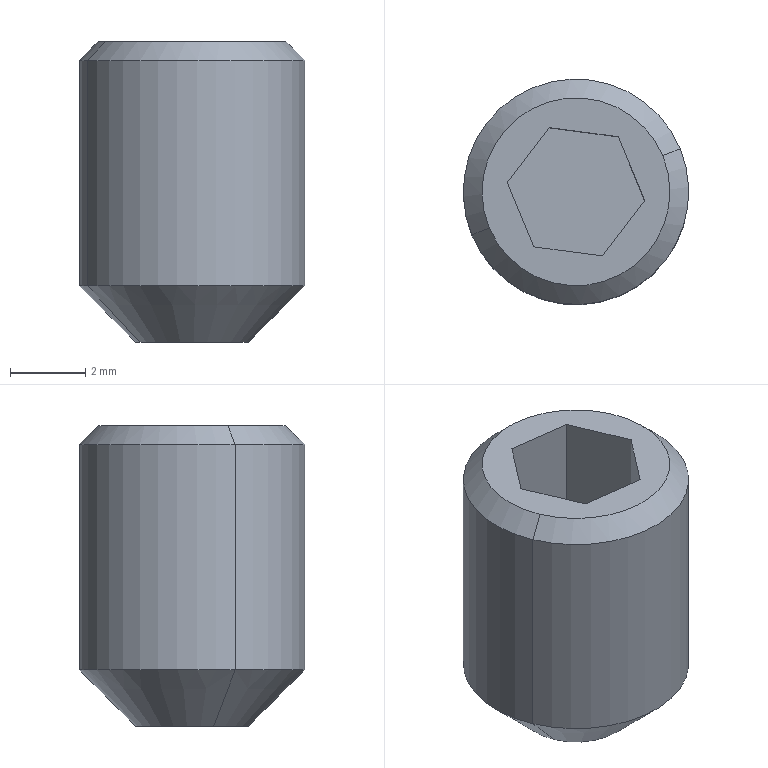Component | SolidWorks | M6x8GrubScrew-3 | 1 solid | 15 faces | box 6 x 6 x 8 mm | volume 171 mm3 | plane 9 | cone 4 | cylinder 2 | commonest cylinder face diameters 6 x2 | material #45
STEP:
#1=COLOUR_RGB('',0.7922,0.8196,0.9333);
#2=FILL_AREA_STYLE_COLOUR('',#1);
#3=FILL_AREA_STYLE('',(#2));
#4=SURFACE_STYLE_FILL_AREA(#3);
#5=SURFACE_SIDE_STYLE('',(#4));
#6=SURFACE_STYLE_USAGE(.BOTH.,#5);
#7=PRESENTATION_STYLE_ASSIGNMENT((#6));
#8=CARTESIAN_POINT('',(-3.53,0.5679,0.4724));
#9=VERTEX_POINT('',#8);
#10=CARTESIAN_POINT('',(-3.421,0.6132,0.4724));
#11=VERTEX_POINT('',#10);
#12=CARTESIAN_POINT('',(-3.476,0.5906,0.4724));
#13=DIRECTION('',(0.,-0.,-1.));
#14=DIRECTION('',(-0.9237,-0.383,0.));
#15=AXIS2_PLACEMENT_3D('',#12,#13,#14);
#16=CIRCLE('',#15,0.05906);
#17=EDGE_CURVE('',#9,#11,#16,.T.);
#18=ORIENTED_EDGE('',*,*,#17,.F.);
#19=CARTESIAN_POINT('',(-3.585,0.5453,0.5315));
#20=VERTEX_POINT('',#19);
#21=CARTESIAN_POINT('',(-3.585,0.5453,0.5315));
#22=DIRECTION('',(-0.6532,-0.2709,0.7071));
#23=VECTOR('',#22,39.37);
#24=LINE('',#21,#23);
#25=EDGE_CURVE('',#9,#20,#24,.T.);
#26=ORIENTED_EDGE('',*,*,#25,.T.);
#27=CARTESIAN_POINT('',(-3.367,0.6358,0.5315));
#28=VERTEX_POINT('',#27);
#29=CARTESIAN_POINT('',(-3.476,0.5906,0.5315));
#30=DIRECTION('',(0.,-0.,-1.));
#31=DIRECTION('',(-0.9237,-0.383,0.));
#32=AXIS2_PLACEMENT_3D('',#29,#30,#31);
#33=CIRCLE('',#32,0.1181);
#34=EDGE_CURVE('',#20,#28,#33,.T.);
#35=ORIENTED_EDGE('',*,*,#34,.T.);
#36=CARTESIAN_POINT('',(-3.367,0.6358,0.5315));
#37=DIRECTION('',(0.6532,0.2709,0.7071));
#38=VECTOR('',#37,39.37);
#39=LINE('',#36,#38);
#40=EDGE_CURVE('',#11,#28,#39,.T.);
#41=ORIENTED_EDGE('',*,*,#40,.F.);
#42=EDGE_LOOP('',(#18,#26,#35,#41));
#43=FACE_OUTER_BOUND('',#42,.T.);
#44=CARTESIAN_POINT('',(-3.476,0.5906,0.5315));
#45=DIRECTION('',(-0.,0.,1.));
#46=DIRECTION('',(0.9237,0.383,0.));
#47=AXIS2_PLACEMENT_3D('',#44,#45,#46);
#48=CONICAL_SURFACE('',#47,0.1181,0.7854);
#49=ADVANCED_FACE('',(#43),#48,.T.);
#50=CARTESIAN_POINT('',(-3.585,0.5453,0.7677));
#51=VERTEX_POINT('',#50);
#52=CARTESIAN_POINT('',(-3.367,0.6358,0.7677));
#53=VERTEX_POINT('',#52);
#54=CARTESIAN_POINT('',(-3.476,0.5906,0.7677));
#55=DIRECTION('',(0.,-0.,-1.));
#56=DIRECTION('',(-0.9237,-0.383,0.));
#57=AXIS2_PLACEMENT_3D('',#54,#55,#56);
#58=CIRCLE('',#57,0.1181);
#59=EDGE_CURVE('',#51,#53,#58,.T.);
#60=ORIENTED_EDGE('',*,*,#59,.T.);
#61=CARTESIAN_POINT('',(-3.367,0.6358,0.4724));
#62=DIRECTION('',(0.,-0.,-1.));
#63=VECTOR('',#62,39.37);
#64=LINE('',#61,#63);
#65=EDGE_CURVE('',#53,#28,#64,.T.);
#66=ORIENTED_EDGE('',*,*,#65,.T.);
#67=ORIENTED_EDGE('',*,*,#34,.F.);
#68=CARTESIAN_POINT('',(-3.585,0.5453,0.4724));
#69=DIRECTION('',(0.,-0.,-1.));
#70=VECTOR('',#69,39.37);
#71=LINE('',#68,#70);
#72=EDGE_CURVE('',#51,#20,#71,.T.);
#73=ORIENTED_EDGE('',*,*,#72,.F.);
#74=EDGE_LOOP('',(#60,#66,#67,#73));
#75=FACE_OUTER_BOUND('',#74,.T.);
#76=CARTESIAN_POINT('',(-3.476,0.5906,0.4724));
#77=DIRECTION('',(0.,-0.,-1.));
#78=DIRECTION('',(-0.9237,-0.383,0.));
#79=AXIS2_PLACEMENT_3D('',#76,#77,#78);
#80=CYLINDRICAL_SURFACE('',#79,0.1181);
#81=ADVANCED_FACE('',(#75),#80,.T.);
#82=CARTESIAN_POINT('',(-3.567,0.5528,0.7874));
#83=VERTEX_POINT('',#82);
#84=CARTESIAN_POINT('',(-3.385,0.6283,0.7874));
#85=VERTEX_POINT('',#84);
#86=CARTESIAN_POINT('',(-3.476,0.5906,0.7874));
#87=DIRECTION('',(0.,-0.,-1.));
#88=DIRECTION('',(-0.9237,-0.383,0.));
#89=AXIS2_PLACEMENT_3D('',#86,#87,#88);
#90=CIRCLE('',#89,0.09843);
#91=EDGE_CURVE('',#83,#85,#90,.T.);
#92=ORIENTED_EDGE('',*,*,#91,.T.);
#93=CARTESIAN_POINT('',(-3.385,0.6283,0.7874));
#94=DIRECTION('',(0.6532,0.2709,-0.7071));
#95=VECTOR('',#94,39.37);
#96=LINE('',#93,#95);
#97=EDGE_CURVE('',#85,#53,#96,.T.);
#98=ORIENTED_EDGE('',*,*,#97,.T.);
#99=ORIENTED_EDGE('',*,*,#59,.F.);
#100=CARTESIAN_POINT('',(-3.567,0.5528,0.7874));
#101=DIRECTION('',(-0.6532,-0.2709,-0.7071));
#102=VECTOR('',#101,39.37);
#103=LINE('',#100,#102);
#104=EDGE_CURVE('',#83,#51,#103,.T.);
#105=ORIENTED_EDGE('',*,*,#104,.F.);
#106=EDGE_LOOP('',(#92,#98,#99,#105));
#107=FACE_OUTER_BOUND('',#106,.T.);
#108=CARTESIAN_POINT('',(-3.476,0.5906,0.7874));
#109=DIRECTION('',(0.,-0.,-1.));
#110=DIRECTION('',(-0.9237,-0.383,0.));
#111=AXIS2_PLACEMENT_3D('',#108,#109,#110);
#112=CONICAL_SURFACE('',#111,0.09843,0.7854);
#113=ADVANCED_FACE('',(#107),#112,.T.);
#114=CARTESIAN_POINT('',(-3.504,0.6577,0.7874));
#115=VERTEX_POINT('',#114);
#116=CARTESIAN_POINT('',(-3.548,0.6,0.7874));
#117=VERTEX_POINT('',#116);
#118=CARTESIAN_POINT('',(-3.504,0.6577,0.7874));
#119=DIRECTION('',(-0.6084,-0.7936,-0.));
#120=VECTOR('',#119,39.37);
#121=LINE('',#118,#120);
#122=EDGE_CURVE('',#115,#117,#121,.T.);
#123=ORIENTED_EDGE('',*,*,#122,.F.);
#124=CARTESIAN_POINT('',(-3.432,0.6483,0.7874));
#125=VERTEX_POINT('',#124);
#126=CARTESIAN_POINT('',(-3.432,0.6483,0.7874));
#127=DIRECTION('',(-0.9915,0.1301,-0.));
#128=VECTOR('',#127,39.37);
#129=LINE('',#126,#128);
#130=EDGE_CURVE('',#125,#115,#129,.T.);
#131=ORIENTED_EDGE('',*,*,#130,.F.);
#132=CARTESIAN_POINT('',(-3.404,0.5811,0.7874));
#133=VERTEX_POINT('',#132);
#134=CARTESIAN_POINT('',(-3.404,0.5811,0.7874));
#135=DIRECTION('',(-0.383,0.9237,-0.));
#136=VECTOR('',#135,39.37);
#137=LINE('',#134,#136);
#138=EDGE_CURVE('',#133,#125,#137,.T.);
#139=ORIENTED_EDGE('',*,*,#138,.F.);
#140=CARTESIAN_POINT('',(-3.448,0.5234,0.7874));
#141=VERTEX_POINT('',#140);
#142=CARTESIAN_POINT('',(-3.448,0.5234,0.7874));
#143=DIRECTION('',(0.6084,0.7936,0.));
#144=VECTOR('',#143,39.37);
#145=LINE('',#142,#144);
#146=EDGE_CURVE('',#141,#133,#145,.T.);
#147=ORIENTED_EDGE('',*,*,#146,.F.);
#148=CARTESIAN_POINT('',(-3.52,0.5328,0.7874));
#149=VERTEX_POINT('',#148);
#150=CARTESIAN_POINT('',(-3.52,0.5328,0.7874));
#151=DIRECTION('',(0.9915,-0.1301,0.));
#152=VECTOR('',#151,39.37);
#153=LINE('',#150,#152);
#154=EDGE_CURVE('',#149,#141,#153,.T.);
#155=ORIENTED_EDGE('',*,*,#154,.F.);
#156=CARTESIAN_POINT('',(-3.548,0.6,0.7874));
#157=DIRECTION('',(0.383,-0.9237,0.));
#158=VECTOR('',#157,39.37);
#159=LINE('',#156,#158);
#160=EDGE_CURVE('',#117,#149,#159,.T.);
#161=ORIENTED_EDGE('',*,*,#160,.F.);
#162=EDGE_LOOP('',(#123,#131,#139,#147,#155,#161));
#163=FACE_BOUND('',#162,.T.);
#164=ORIENTED_EDGE('',*,*,#91,.F.);
#165=CARTESIAN_POINT('',(-3.476,0.5906,0.7874));
#166=DIRECTION('',(0.,-0.,-1.));
#167=DIRECTION('',(-0.9237,-0.383,0.));
#168=AXIS2_PLACEMENT_3D('',#165,#166,#167);
#169=CIRCLE('',#168,0.09843);
#170=EDGE_CURVE('',#85,#83,#169,.T.);
#171=ORIENTED_EDGE('',*,*,#170,.F.);
#172=EDGE_LOOP('',(#164,#171));
#173=FACE_OUTER_BOUND('',#172,.T.);
#174=CARTESIAN_POINT('',(-3.476,0.5906,0.7874));
#175=DIRECTION('',(0.,-0.,-1.));
#176=DIRECTION('',(-0.9237,-0.383,-0.));
#177=AXIS2_PLACEMENT_3D('',#174,#175,#176);
#178=PLANE('',#177);
#179=ADVANCED_FACE('',(#163,#173),#178,.F.);
#180=ORIENTED_EDGE('',*,*,#97,.F.);
#181=ORIENTED_EDGE('',*,*,#170,.T.);
#182=ORIENTED_EDGE('',*,*,#104,.T.);
#183=CARTESIAN_POINT('',(-3.476,0.5906,0.7677));
#184=DIRECTION('',(0.,-0.,-1.));
#185=DIRECTION('',(-0.9237,-0.383,0.));
#186=AXIS2_PLACEMENT_3D('',#183,#184,#185);
#187=CIRCLE('',#186,0.1181);
#188=EDGE_CURVE('',#53,#51,#187,.T.);
#189=ORIENTED_EDGE('',*,*,#188,.F.);
#190=EDGE_LOOP('',(#180,#181,#182,#189));
#191=FACE_OUTER_BOUND('',#190,.T.);
#192=CARTESIAN_POINT('',(-3.476,0.5906,0.7874));
#193=DIRECTION('',(0.,-0.,-1.));
#194=DIRECTION('',(-0.9237,-0.383,0.));
#195=AXIS2_PLACEMENT_3D('',#192,#193,#194);
#196=CONICAL_SURFACE('',#195,0.09843,0.7854);
#197=ADVANCED_FACE('',(#191),#196,.T.);
#198=ORIENTED_EDGE('',*,*,#65,.F.);
#199=ORIENTED_EDGE('',*,*,#188,.T.);
#200=ORIENTED_EDGE('',*,*,#72,.T.);
#201=CARTESIAN_POINT('',(-3.476,0.5906,0.5315));
#202=DIRECTION('',(0.,-0.,-1.));
#203=DIRECTION('',(-0.9237,-0.383,0.));
#204=AXIS2_PLACEMENT_3D('',#201,#202,#203);
#205=CIRCLE('',#204,0.1181);
#206=EDGE_CURVE('',#28,#20,#205,.T.);
#207=ORIENTED_EDGE('',*,*,#206,.F.);
#208=EDGE_LOOP('',(#198,#199,#200,#207));
#209=FACE_OUTER_BOUND('',#208,.T.);
#210=CARTESIAN_POINT('',(-3.476,0.5906,0.4724));
#211=DIRECTION('',(0.,-0.,-1.));
#212=DIRECTION('',(-0.9237,-0.383,0.));
#213=AXIS2_PLACEMENT_3D('',#210,#211,#212);
#214=CYLINDRICAL_SURFACE('',#213,0.1181);
#215=ADVANCED_FACE('',(#209),#214,.T.);
#216=ORIENTED_EDGE('',*,*,#25,.F.);
#217=CARTESIAN_POINT('',(-3.476,0.5906,0.4724));
#218=DIRECTION('',(0.,-0.,-1.));
#219=DIRECTION('',(-0.9237,-0.383,0.));
#220=AXIS2_PLACEMENT_3D('',#217,#218,#219);
#221=CIRCLE('',#220,0.05906);
#222=EDGE_CURVE('',#11,#9,#221,.T.);
#223=ORIENTED_EDGE('',*,*,#222,.F.);
#224=ORIENTED_EDGE('',*,*,#40,.T.);
#225=ORIENTED_EDGE('',*,*,#206,.T.);
#226=EDGE_LOOP('',(#216,#223,#224,#225));
#227=FACE_OUTER_BOUND('',#226,.T.);
#228=CARTESIAN_POINT('',(-3.476,0.5906,0.5315));
#229=DIRECTION('',(-0.,0.,1.));
#230=DIRECTION('',(0.9237,0.383,0.));
#231=AXIS2_PLACEMENT_3D('',#228,#229,#230);
#232=CONICAL_SURFACE('',#231,0.1181,0.7854);
#233=ADVANCED_FACE('',(#227),#232,.T.);
#234=ORIENTED_EDGE('',*,*,#222,.T.);
#235=ORIENTED_EDGE('',*,*,#17,.T.);
#236=EDGE_LOOP('',(#234,#235));
#237=FACE_OUTER_BOUND('',#236,.T.);
#238=CARTESIAN_POINT('',(-3.421,0.6132,0.4724));
#239=DIRECTION('',(-0.,0.,1.));
#240=DIRECTION('',(0.9237,0.383,0.));
#241=AXIS2_PLACEMENT_3D('',#238,#239,#240);
#242=PLANE('',#241);
#243=ADVANCED_FACE('',(#237),#242,.F.);
#244=ORIENTED_EDGE('',*,*,#130,.T.);
#245=CARTESIAN_POINT('',(-3.504,0.6577,0.6299));
#246=VERTEX_POINT('',#245);
#247=CARTESIAN_POINT('',(-3.504,0.6577,0.6299));
#248=DIRECTION('',(-0.,0.,1.));
#249=VECTOR('',#248,39.37);
#250=LINE('',#247,#249);
#251=EDGE_CURVE('',#246,#115,#250,.T.);
#252=ORIENTED_EDGE('',*,*,#251,.F.);
#253=CARTESIAN_POINT('',(-3.432,0.6483,0.6299));
#254=VERTEX_POINT('',#253);
#255=CARTESIAN_POINT('',(-3.432,0.6483,0.6299));
#256=DIRECTION('',(-0.9915,0.1301,-0.));
#257=VECTOR('',#256,39.37);
#258=LINE('',#255,#257);
#259=EDGE_CURVE('',#254,#246,#258,.T.);
#260=ORIENTED_EDGE('',*,*,#259,.F.);
#261=CARTESIAN_POINT('',(-3.432,0.6483,0.6299));
#262=DIRECTION('',(-0.,0.,1.));
#263=VECTOR('',#262,39.37);
#264=LINE('',#261,#263);
#265=EDGE_CURVE('',#254,#125,#264,.T.);
#266=ORIENTED_EDGE('',*,*,#265,.T.);
#267=EDGE_LOOP('',(#244,#252,#260,#266));
#268=FACE_OUTER_BOUND('',#267,.T.);
#269=CARTESIAN_POINT('',(-3.432,0.6483,0.6299));
#270=DIRECTION('',(0.1301,0.9915,-0.));
#271=DIRECTION('',(0.9915,-0.1301,0.));
#272=AXIS2_PLACEMENT_3D('',#269,#270,#271);
#273=PLANE('',#272);
#274=ADVANCED_FACE('',(#268),#273,.F.);
#275=ORIENTED_EDGE('',*,*,#138,.T.);
#276=ORIENTED_EDGE('',*,*,#265,.F.);
#277=CARTESIAN_POINT('',(-3.404,0.5811,0.6299));
#278=VERTEX_POINT('',#277);
#279=CARTESIAN_POINT('',(-3.404,0.5811,0.6299));
#280=DIRECTION('',(-0.383,0.9237,-0.));
#281=VECTOR('',#280,39.37);
#282=LINE('',#279,#281);
#283=EDGE_CURVE('',#278,#254,#282,.T.);
#284=ORIENTED_EDGE('',*,*,#283,.F.);
#285=CARTESIAN_POINT('',(-3.404,0.5811,0.6299));
#286=DIRECTION('',(-0.,0.,1.));
#287=VECTOR('',#286,39.37);
#288=LINE('',#285,#287);
#289=EDGE_CURVE('',#278,#133,#288,.T.);
#290=ORIENTED_EDGE('',*,*,#289,.T.);
#291=EDGE_LOOP('',(#275,#276,#284,#290));
#292=FACE_OUTER_BOUND('',#291,.T.);
#293=CARTESIAN_POINT('',(-3.404,0.5811,0.6299));
#294=DIRECTION('',(0.9237,0.383,0.));
#295=DIRECTION('',(0.383,-0.9237,0.));
#296=AXIS2_PLACEMENT_3D('',#293,#294,#295);
#297=PLANE('',#296);
#298=ADVANCED_FACE('',(#292),#297,.F.);
#299=ORIENTED_EDGE('',*,*,#146,.T.);
#300=ORIENTED_EDGE('',*,*,#289,.F.);
#301=CARTESIAN_POINT('',(-3.448,0.5234,0.6299));
#302=VERTEX_POINT('',#301);
#303=CARTESIAN_POINT('',(-3.448,0.5234,0.6299));
#304=DIRECTION('',(0.6084,0.7936,0.));
#305=VECTOR('',#304,39.37);
#306=LINE('',#303,#305);
#307=EDGE_CURVE('',#302,#278,#306,.T.);
#308=ORIENTED_EDGE('',*,*,#307,.F.);
#309=CARTESIAN_POINT('',(-3.448,0.5234,0.6299));
#310=DIRECTION('',(-0.,0.,1.));
#311=VECTOR('',#310,39.37);
#312=LINE('',#309,#311);
#313=EDGE_CURVE('',#302,#141,#312,.T.);
#314=ORIENTED_EDGE('',*,*,#313,.T.);
#315=EDGE_LOOP('',(#299,#300,#308,#314));
#316=FACE_OUTER_BOUND('',#315,.T.);
#317=CARTESIAN_POINT('',(-3.448,0.5234,0.6299));
#318=DIRECTION('',(0.7936,-0.6084,0.));
#319=DIRECTION('',(-0.6084,-0.7936,-0.));
#320=AXIS2_PLACEMENT_3D('',#317,#318,#319);
#321=PLANE('',#320);
#322=ADVANCED_FACE('',(#316),#321,.F.);
#323=ORIENTED_EDGE('',*,*,#154,.T.);
#324=ORIENTED_EDGE('',*,*,#313,.F.);
#325=CARTESIAN_POINT('',(-3.52,0.5328,0.6299));
#326=VERTEX_POINT('',#325);
#327=CARTESIAN_POINT('',(-3.52,0.5328,0.6299));
#328=DIRECTION('',(0.9915,-0.1301,0.));
#329=VECTOR('',#328,39.37);
#330=LINE('',#327,#329);
#331=EDGE_CURVE('',#326,#302,#330,.T.);
#332=ORIENTED_EDGE('',*,*,#331,.F.);
#333=CARTESIAN_POINT('',(-3.52,0.5328,0.6299));
#334=DIRECTION('',(-0.,0.,1.));
#335=VECTOR('',#334,39.37);
#336=LINE('',#333,#335);
#337=EDGE_CURVE('',#326,#149,#336,.T.);
#338=ORIENTED_EDGE('',*,*,#337,.T.);
#339=EDGE_LOOP('',(#323,#324,#332,#338));
#340=FACE_OUTER_BOUND('',#339,.T.);
#341=CARTESIAN_POINT('',(-3.52,0.5328,0.6299));
#342=DIRECTION('',(-0.1301,-0.9915,0.));
#343=DIRECTION('',(-0.9915,0.1301,-0.));
#344=AXIS2_PLACEMENT_3D('',#341,#342,#343);
#345=PLANE('',#344);
#346=ADVANCED_FACE('',(#340),#345,.F.);
#347=ORIENTED_EDGE('',*,*,#160,.T.);
#348=ORIENTED_EDGE('',*,*,#337,.F.);
#349=CARTESIAN_POINT('',(-3.548,0.6,0.6299));
#350=VERTEX_POINT('',#349);
#351=CARTESIAN_POINT('',(-3.548,0.6,0.6299));
#352=DIRECTION('',(0.383,-0.9237,0.));
#353=VECTOR('',#352,39.37);
#354=LINE('',#351,#353);
#355=EDGE_CURVE('',#350,#326,#354,.T.);
#356=ORIENTED_EDGE('',*,*,#355,.F.);
#357=CARTESIAN_POINT('',(-3.548,0.6,0.6299));
#358=DIRECTION('',(-0.,0.,1.));
#359=VECTOR('',#358,39.37);
#360=LINE('',#357,#359);
#361=EDGE_CURVE('',#350,#117,#360,.T.);
#362=ORIENTED_EDGE('',*,*,#361,.T.);
#363=EDGE_LOOP('',(#347,#348,#356,#362));
#364=FACE_OUTER_BOUND('',#363,.T.);
#365=CARTESIAN_POINT('',(-3.548,0.6,0.6299));
#366=DIRECTION('',(-0.9237,-0.383,-0.));
#367=DIRECTION('',(-0.,0.,1.));
#368=AXIS2_PLACEMENT_3D('',#365,#366,#367);
#369=PLANE('',#368);
#370=ADVANCED_FACE('',(#364),#369,.F.);
#371=ORIENTED_EDGE('',*,*,#122,.T.);
#372=ORIENTED_EDGE('',*,*,#361,.F.);
#373=CARTESIAN_POINT('',(-3.504,0.6577,0.6299));
#374=DIRECTION('',(-0.6084,-0.7936,-0.));
#375=VECTOR('',#374,39.37);
#376=LINE('',#373,#375);
#377=EDGE_CURVE('',#246,#350,#376,.T.);
#378=ORIENTED_EDGE('',*,*,#377,.F.);
#379=ORIENTED_EDGE('',*,*,#251,.T.);
#380=EDGE_LOOP('',(#371,#372,#378,#379));
#381=FACE_OUTER_BOUND('',#380,.T.);
#382=CARTESIAN_POINT('',(-3.504,0.6577,0.6299));
#383=DIRECTION('',(-0.7936,0.6084,-0.));
#384=DIRECTION('',(0.6084,0.7936,0.));
#385=AXIS2_PLACEMENT_3D('',#382,#383,#384);
#386=PLANE('',#385);
#387=ADVANCED_FACE('',(#381),#386,.F.);
#388=ORIENTED_EDGE('',*,*,#259,.T.);
#389=ORIENTED_EDGE('',*,*,#377,.T.);
#390=ORIENTED_EDGE('',*,*,#355,.T.);
#391=ORIENTED_EDGE('',*,*,#331,.T.);
#392=ORIENTED_EDGE('',*,*,#307,.T.);
#393=ORIENTED_EDGE('',*,*,#283,.T.);
#394=EDGE_LOOP('',(#388,#389,#390,#391,#392,#393));
#395=FACE_OUTER_BOUND('',#394,.T.);
#396=CARTESIAN_POINT('',(-3.476,0.5906,0.6299));
#397=DIRECTION('',(-0.,0.,1.));
#398=DIRECTION('',(0.9237,0.383,0.));
#399=AXIS2_PLACEMENT_3D('',#396,#397,#398);
#400=PLANE('',#399);
#401=ADVANCED_FACE('',(#395),#400,.T.);
#402=CLOSED_SHELL('',(#49,#81,#113,#179,#197,#215,#233,#243,#274,#298,#322,#346,#370,#387,#401));
#403=MANIFOLD_SOLID_BREP('',#402);
#404=STYLED_ITEM('',(#7),#403);
#405=(LENGTH_UNIT()NAMED_UNIT(*)SI_UNIT($,.METRE.));
#406=LENGTH_MEASURE_WITH_UNIT(LENGTH_MEASURE(0.0254),#405);
#407=DIMENSIONAL_EXPONENTS(1.,0.,0.,0.,0.,0.,0.);
#408=(CONVERSION_BASED_UNIT('',#406)LENGTH_UNIT()NAMED_UNIT(#407));
#409=UNCERTAINTY_MEASURE_WITH_UNIT(LENGTH_MEASURE(0.00001),#408,'','');
#410=(NAMED_UNIT(*)PLANE_ANGLE_UNIT()SI_UNIT($,.RADIAN.));
#411=(NAMED_UNIT(*)SI_UNIT($,.STERADIAN.)SOLID_ANGLE_UNIT());
#412=(GEOMETRIC_REPRESENTATION_CONTEXT(3)GLOBAL_UNCERTAINTY_ASSIGNED_CONTEXT((#409))GLOBAL_UNIT_ASSIGNED_CONTEXT((#408,#410,#411))REPRESENTATION_CONTEXT('',''));
#413=MECHANICAL_DESIGN_GEOMETRIC_PRESENTATION_REPRESENTATION('',(#404),#412);
#414=CARTESIAN_POINT('',(0.,0.,0.));
#415=DIRECTION('',(0.,0.,1.));
#416=DIRECTION('',(1.,0.,0.));
#417=AXIS2_PLACEMENT_3D('',#414,#415,#416);
#418=(LENGTH_UNIT()NAMED_UNIT(*)SI_UNIT($,.METRE.));
#419=LENGTH_MEASURE_WITH_UNIT(LENGTH_MEASURE(0.0254),#418);
#420=DIMENSIONAL_EXPONENTS(1.,0.,0.,0.,0.,0.,0.);
#421=(CONVERSION_BASED_UNIT('',#419)LENGTH_UNIT()NAMED_UNIT(#420));
#422=UNCERTAINTY_MEASURE_WITH_UNIT(LENGTH_MEASURE(0.00001),#421,'','');
#423=(NAMED_UNIT(*)PLANE_ANGLE_UNIT()SI_UNIT($,.RADIAN.));
#424=(NAMED_UNIT(*)SI_UNIT($,.STERADIAN.)SOLID_ANGLE_UNIT());
#425=(GEOMETRIC_REPRESENTATION_CONTEXT(3)GLOBAL_UNCERTAINTY_ASSIGNED_CONTEXT((#422))GLOBAL_UNIT_ASSIGNED_CONTEXT((#421,#423,#424))REPRESENTATION_CONTEXT('',''));
#426=ADVANCED_BREP_SHAPE_REPRESENTATION('',(#403,#417),#425);
#427=PRESENTATION_LAYER_ASSIGNMENT('','',(#404));